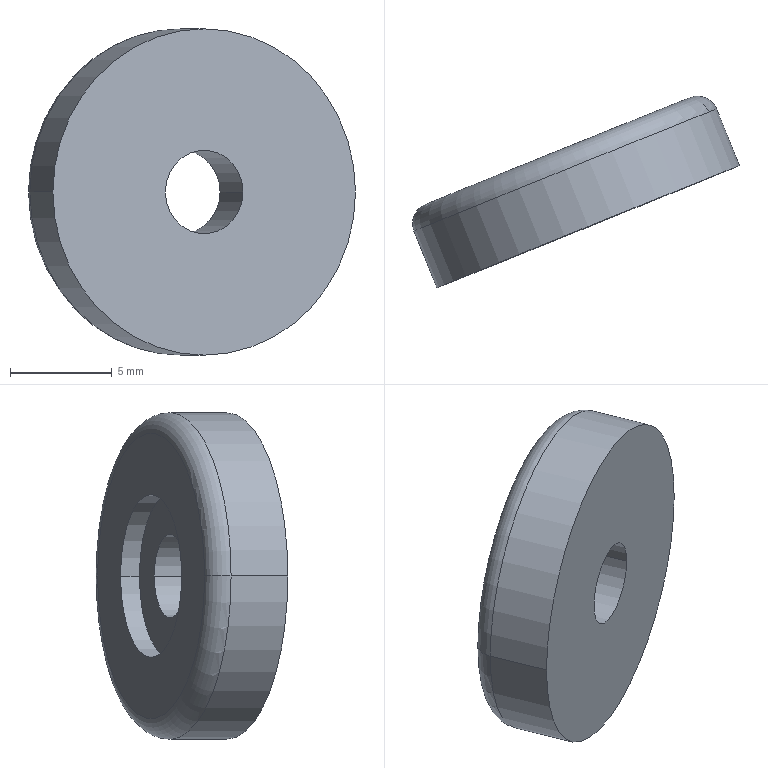Component | SolidWorks | RightDoorAssembly-1_LinkRodLock-1_Roller-4 | 1 solid | 11 faces | box 16.03 x 9.4 x 16 mm | volume 704 mm3 | cylinder 6 | plane 3 | torus 2 | commonest cylinder face diameters 8 x2 16 x2 4.1 x2
build123d program:
from build123d import *

# Parameters (mm, degrees)
SKETCH1_R           = 8
SKETCH1_R_2         = 2.05
BOSS_EXTRUDE1_DEPTH = 4
SKETCH2_R           = 4
CUT_EXTRUDE1_DEPTH  = 1
FILLET1_R           = 1


with BuildPart() as part:
    # Sketch1 → Boss-Extrude1 (new body)
    with BuildSketch(Plane.XY):
        Circle(SKETCH1_R)
        Circle(SKETCH1_R_2, mode=Mode.SUBTRACT)
    extrude(amount=BOSS_EXTRUDE1_DEPTH)

    # Sketch2 → Cut-Extrude1 (cut)
    with BuildSketch(Plane.XY.offset(4)):
        Circle(SKETCH2_R)
    extrude(amount=-CUT_EXTRUDE1_DEPTH, mode=Mode.SUBTRACT)

    # Fillet1
    fillet1_edges = [part.edges().sort_by_distance(p)[0] for p in [
        (-8, 0, 4),
    ]]
    fillet(fillet1_edges, radius=FILLET1_R)


solid = part.part

# Placed as in the assembly
solid = solid.moved(Location((-316.148, 410.532, 94.7), (-90, -21.985, 6.077)))
STEP:
#1=COLOUR_RGB('',0.7922,0.8196,0.9333);
#2=FILL_AREA_STYLE_COLOUR('',#1);
#3=FILL_AREA_STYLE('',(#2));
#4=SURFACE_STYLE_FILL_AREA(#3);
#5=SURFACE_SIDE_STYLE('',(#4));
#6=SURFACE_STYLE_USAGE(.BOTH.,#5);
#7=PRESENTATION_STYLE_ASSIGNMENT((#6));
#8=CARTESIAN_POINT('',(-12.199,16.39,3.728));
#9=VERTEX_POINT('',#8);
#10=CARTESIAN_POINT('',(-12.783,16.154,3.728));
#11=VERTEX_POINT('',#10);
#12=CARTESIAN_POINT('',(-12.491,16.272,3.728));
#13=DIRECTION('',(0.3744,-0.9273,0.));
#14=DIRECTION('',(-0.9273,-0.3744,0.));
#15=AXIS2_PLACEMENT_3D('',#12,#13,#14);
#16=CIRCLE('',#15,0.315);
#17=EDGE_CURVE('',#9,#11,#16,.T.);
#18=ORIENTED_EDGE('',*,*,#17,.F.);
#19=CARTESIAN_POINT('',(-12.25,16.412,3.728));
#20=VERTEX_POINT('',#19);
#21=CARTESIAN_POINT('',(-12.235,16.375,3.728));
#22=DIRECTION('',(0.,0.,1.));
#23=DIRECTION('',(0.,-1.,0.));
#24=AXIS2_PLACEMENT_3D('',#21,#22,#23);
#25=CIRCLE('',#24,0.03937);
#26=EDGE_CURVE('',#9,#20,#25,.T.);
#27=ORIENTED_EDGE('',*,*,#26,.T.);
#28=CARTESIAN_POINT('',(-12.761,16.206,3.728));
#29=VERTEX_POINT('',#28);
#30=CARTESIAN_POINT('',(-12.506,16.309,3.728));
#31=DIRECTION('',(-0.3744,0.9273,-0.));
#32=DIRECTION('',(-0.9273,-0.3744,0.));
#33=AXIS2_PLACEMENT_3D('',#30,#31,#32);
#34=CIRCLE('',#33,0.2756);
#35=EDGE_CURVE('',#29,#20,#34,.T.);
#36=ORIENTED_EDGE('',*,*,#35,.F.);
#37=CARTESIAN_POINT('',(-12.747,16.169,3.728));
#38=DIRECTION('',(-0.,-0.,-1.));
#39=DIRECTION('',(0.,1.,-0.));
#40=AXIS2_PLACEMENT_3D('',#37,#38,#39);
#41=CIRCLE('',#40,0.03937);
#42=EDGE_CURVE('',#11,#29,#41,.T.);
#43=ORIENTED_EDGE('',*,*,#42,.F.);
#44=EDGE_LOOP('',(#18,#27,#36,#43));
#45=FACE_OUTER_BOUND('',#44,.T.);
#46=CARTESIAN_POINT('',(-12.491,16.272,3.728));
#47=DIRECTION('',(-0.3744,0.9273,-0.));
#48=DIRECTION('',(-0.9273,-0.3744,0.));
#49=AXIS2_PLACEMENT_3D('',#46,#47,#48);
#50=TOROIDAL_SURFACE('',#49,0.2756,0.03937);
#51=ADVANCED_FACE('',(#45),#50,.T.);
#52=CARTESIAN_POINT('',(-12.345,16.331,3.728));
#53=VERTEX_POINT('',#52);
#54=CARTESIAN_POINT('',(-12.637,16.213,3.728));
#55=VERTEX_POINT('',#54);
#56=CARTESIAN_POINT('',(-12.491,16.272,3.728));
#57=DIRECTION('',(-0.3744,0.9273,-0.));
#58=DIRECTION('',(-0.9273,-0.3744,0.));
#59=AXIS2_PLACEMENT_3D('',#56,#57,#58);
#60=CIRCLE('',#59,0.1575);
#61=EDGE_CURVE('',#53,#55,#60,.T.);
#62=ORIENTED_EDGE('',*,*,#61,.F.);
#63=CARTESIAN_POINT('',(-12.36,16.368,3.728));
#64=VERTEX_POINT('',#63);
#65=CARTESIAN_POINT('',(-12.345,16.331,3.728));
#66=DIRECTION('',(-0.3744,0.9273,-0.));
#67=VECTOR('',#66,39.37);
#68=LINE('',#65,#67);
#69=EDGE_CURVE('',#53,#64,#68,.T.);
#70=ORIENTED_EDGE('',*,*,#69,.T.);
#71=CARTESIAN_POINT('',(-12.652,16.25,3.728));
#72=VERTEX_POINT('',#71);
#73=CARTESIAN_POINT('',(-12.506,16.309,3.728));
#74=DIRECTION('',(-0.3744,0.9273,-0.));
#75=DIRECTION('',(-0.9273,-0.3744,0.));
#76=AXIS2_PLACEMENT_3D('',#73,#74,#75);
#77=CIRCLE('',#76,0.1575);
#78=EDGE_CURVE('',#64,#72,#77,.T.);
#79=ORIENTED_EDGE('',*,*,#78,.T.);
#80=CARTESIAN_POINT('',(-12.637,16.213,3.728));
#81=DIRECTION('',(-0.3744,0.9273,-0.));
#82=VECTOR('',#81,39.37);
#83=LINE('',#80,#82);
#84=EDGE_CURVE('',#55,#72,#83,.T.);
#85=ORIENTED_EDGE('',*,*,#84,.F.);
#86=EDGE_LOOP('',(#62,#70,#79,#85));
#87=FACE_OUTER_BOUND('',#86,.T.);
#88=CARTESIAN_POINT('',(-12.491,16.272,3.728));
#89=DIRECTION('',(-0.3744,0.9273,-0.));
#90=DIRECTION('',(-0.9273,-0.3744,0.));
#91=AXIS2_PLACEMENT_3D('',#88,#89,#90);
#92=CYLINDRICAL_SURFACE('',#91,0.1575);
#93=ADVANCED_FACE('',(#87),#92,.F.);
#94=ORIENTED_EDGE('',*,*,#17,.T.);
#95=CARTESIAN_POINT('',(-12.739,16.045,3.728));
#96=VERTEX_POINT('',#95);
#97=CARTESIAN_POINT('',(-12.798,16.191,3.728));
#98=DIRECTION('',(0.3744,-0.9273,0.));
#99=VECTOR('',#98,39.37);
#100=LINE('',#97,#99);
#101=EDGE_CURVE('',#11,#96,#100,.T.);
#102=ORIENTED_EDGE('',*,*,#101,.T.);
#103=CARTESIAN_POINT('',(-12.155,16.281,3.728));
#104=VERTEX_POINT('',#103);
#105=CARTESIAN_POINT('',(-12.447,16.163,3.728));
#106=DIRECTION('',(-0.3744,0.9273,-0.));
#107=DIRECTION('',(-0.9273,-0.3744,0.));
#108=AXIS2_PLACEMENT_3D('',#105,#106,#107);
#109=CIRCLE('',#108,0.315);
#110=EDGE_CURVE('',#96,#104,#109,.T.);
#111=ORIENTED_EDGE('',*,*,#110,.T.);
#112=CARTESIAN_POINT('',(-12.214,16.427,3.728));
#113=DIRECTION('',(0.3744,-0.9273,0.));
#114=VECTOR('',#113,39.37);
#115=LINE('',#112,#114);
#116=EDGE_CURVE('',#9,#104,#115,.T.);
#117=ORIENTED_EDGE('',*,*,#116,.F.);
#118=EDGE_LOOP('',(#94,#102,#111,#117));
#119=FACE_OUTER_BOUND('',#118,.T.);
#120=CARTESIAN_POINT('',(-12.506,16.309,3.728));
#121=DIRECTION('',(0.3744,-0.9273,0.));
#122=DIRECTION('',(0.9273,0.3744,-0.));
#123=AXIS2_PLACEMENT_3D('',#120,#121,#122);
#124=CYLINDRICAL_SURFACE('',#123,0.315);
#125=ADVANCED_FACE('',(#119),#124,.T.);
#126=CARTESIAN_POINT('',(-12.416,16.302,3.728));
#127=VERTEX_POINT('',#126);
#128=CARTESIAN_POINT('',(-12.566,16.242,3.728));
#129=VERTEX_POINT('',#128);
#130=CARTESIAN_POINT('',(-12.491,16.272,3.728));
#131=DIRECTION('',(-0.3744,0.9273,-0.));
#132=DIRECTION('',(-0.9273,-0.3744,0.));
#133=AXIS2_PLACEMENT_3D('',#130,#131,#132);
#134=CIRCLE('',#133,0.08071);
#135=EDGE_CURVE('',#127,#129,#134,.T.);
#136=ORIENTED_EDGE('',*,*,#135,.T.);
#137=CARTESIAN_POINT('',(-12.522,16.132,3.728));
#138=VERTEX_POINT('',#137);
#139=CARTESIAN_POINT('',(-12.581,16.278,3.728));
#140=DIRECTION('',(0.3744,-0.9273,0.));
#141=VECTOR('',#140,39.37);
#142=LINE('',#139,#141);
#143=EDGE_CURVE('',#129,#138,#142,.T.);
#144=ORIENTED_EDGE('',*,*,#143,.T.);
#145=CARTESIAN_POINT('',(-12.372,16.193,3.728));
#146=VERTEX_POINT('',#145);
#147=CARTESIAN_POINT('',(-12.447,16.163,3.728));
#148=DIRECTION('',(-0.3744,0.9273,-0.));
#149=DIRECTION('',(-0.9273,-0.3744,0.));
#150=AXIS2_PLACEMENT_3D('',#147,#148,#149);
#151=CIRCLE('',#150,0.08071);
#152=EDGE_CURVE('',#146,#138,#151,.T.);
#153=ORIENTED_EDGE('',*,*,#152,.F.);
#154=CARTESIAN_POINT('',(-12.431,16.339,3.728));
#155=DIRECTION('',(0.3744,-0.9273,0.));
#156=VECTOR('',#155,39.37);
#157=LINE('',#154,#156);
#158=EDGE_CURVE('',#127,#146,#157,.T.);
#159=ORIENTED_EDGE('',*,*,#158,.F.);
#160=EDGE_LOOP('',(#136,#144,#153,#159));
#161=FACE_OUTER_BOUND('',#160,.T.);
#162=CARTESIAN_POINT('',(-12.506,16.309,3.728));
#163=DIRECTION('',(0.3744,-0.9273,0.));
#164=DIRECTION('',(0.9273,0.3744,-0.));
#165=AXIS2_PLACEMENT_3D('',#162,#163,#164);
#166=CYLINDRICAL_SURFACE('',#165,0.08071);
#167=ADVANCED_FACE('',(#161),#166,.F.);
#168=ORIENTED_EDGE('',*,*,#143,.F.);
#169=CARTESIAN_POINT('',(-12.491,16.272,3.728));
#170=DIRECTION('',(-0.3744,0.9273,-0.));
#171=DIRECTION('',(-0.9273,-0.3744,0.));
#172=AXIS2_PLACEMENT_3D('',#169,#170,#171);
#173=CIRCLE('',#172,0.08071);
#174=EDGE_CURVE('',#129,#127,#173,.T.);
#175=ORIENTED_EDGE('',*,*,#174,.T.);
#176=ORIENTED_EDGE('',*,*,#158,.T.);
#177=CARTESIAN_POINT('',(-12.447,16.163,3.728));
#178=DIRECTION('',(-0.3744,0.9273,-0.));
#179=DIRECTION('',(-0.9273,-0.3744,0.));
#180=AXIS2_PLACEMENT_3D('',#177,#178,#179);
#181=CIRCLE('',#180,0.08071);
#182=EDGE_CURVE('',#138,#146,#181,.T.);
#183=ORIENTED_EDGE('',*,*,#182,.F.);
#184=EDGE_LOOP('',(#168,#175,#176,#183));
#185=FACE_OUTER_BOUND('',#184,.T.);
#186=CARTESIAN_POINT('',(-12.506,16.309,3.728));
#187=DIRECTION('',(0.3744,-0.9273,0.));
#188=DIRECTION('',(0.9273,0.3744,-0.));
#189=AXIS2_PLACEMENT_3D('',#186,#187,#188);
#190=CYLINDRICAL_SURFACE('',#189,0.08071);
#191=ADVANCED_FACE('',(#185),#190,.F.);
#192=ORIENTED_EDGE('',*,*,#35,.T.);
#193=CARTESIAN_POINT('',(-12.506,16.309,3.728));
#194=DIRECTION('',(-0.3744,0.9273,-0.));
#195=DIRECTION('',(-0.9273,-0.3744,0.));
#196=AXIS2_PLACEMENT_3D('',#193,#194,#195);
#197=CIRCLE('',#196,0.2756);
#198=EDGE_CURVE('',#20,#29,#197,.T.);
#199=ORIENTED_EDGE('',*,*,#198,.T.);
#200=EDGE_LOOP('',(#192,#199));
#201=FACE_OUTER_BOUND('',#200,.T.);
#202=CARTESIAN_POINT('',(-12.506,16.309,3.728));
#203=DIRECTION('',(-0.3744,0.9273,-0.));
#204=DIRECTION('',(-0.9273,-0.3744,0.));
#205=AXIS2_PLACEMENT_3D('',#202,#203,#204);
#206=CIRCLE('',#205,0.1575);
#207=EDGE_CURVE('',#72,#64,#206,.T.);
#208=ORIENTED_EDGE('',*,*,#207,.F.);
#209=ORIENTED_EDGE('',*,*,#78,.F.);
#210=EDGE_LOOP('',(#208,#209));
#211=FACE_BOUND('',#210,.T.);
#212=CARTESIAN_POINT('',(-12.506,16.309,3.728));
#213=DIRECTION('',(-0.3744,0.9273,-0.));
#214=DIRECTION('',(-0.9273,-0.3744,0.));
#215=AXIS2_PLACEMENT_3D('',#212,#213,#214);
#216=PLANE('',#215);
#217=ADVANCED_FACE('',(#201,#211),#216,.T.);
#218=CARTESIAN_POINT('',(-12.447,16.163,3.728));
#219=DIRECTION('',(-0.3744,0.9273,-0.));
#220=DIRECTION('',(-0.9273,-0.3744,0.));
#221=AXIS2_PLACEMENT_3D('',#218,#219,#220);
#222=CIRCLE('',#221,0.315);
#223=EDGE_CURVE('',#104,#96,#222,.T.);
#224=ORIENTED_EDGE('',*,*,#223,.F.);
#225=ORIENTED_EDGE('',*,*,#110,.F.);
#226=EDGE_LOOP('',(#224,#225));
#227=FACE_OUTER_BOUND('',#226,.T.);
#228=ORIENTED_EDGE('',*,*,#152,.T.);
#229=ORIENTED_EDGE('',*,*,#182,.T.);
#230=EDGE_LOOP('',(#228,#229));
#231=FACE_BOUND('',#230,.T.);
#232=CARTESIAN_POINT('',(-12.447,16.163,3.728));
#233=DIRECTION('',(-0.3744,0.9273,-0.));
#234=DIRECTION('',(-0.9273,-0.3744,0.));
#235=AXIS2_PLACEMENT_3D('',#232,#233,#234);
#236=PLANE('',#235);
#237=ADVANCED_FACE('',(#227,#231),#236,.F.);
#238=ORIENTED_EDGE('',*,*,#101,.F.);
#239=CARTESIAN_POINT('',(-12.491,16.272,3.728));
#240=DIRECTION('',(0.3744,-0.9273,0.));
#241=DIRECTION('',(-0.9273,-0.3744,0.));
#242=AXIS2_PLACEMENT_3D('',#239,#240,#241);
#243=CIRCLE('',#242,0.315);
#244=EDGE_CURVE('',#11,#9,#243,.T.);
#245=ORIENTED_EDGE('',*,*,#244,.T.);
#246=ORIENTED_EDGE('',*,*,#116,.T.);
#247=ORIENTED_EDGE('',*,*,#223,.T.);
#248=EDGE_LOOP('',(#238,#245,#246,#247));
#249=FACE_OUTER_BOUND('',#248,.T.);
#250=CARTESIAN_POINT('',(-12.506,16.309,3.728));
#251=DIRECTION('',(0.3744,-0.9273,0.));
#252=DIRECTION('',(0.9273,0.3744,-0.));
#253=AXIS2_PLACEMENT_3D('',#250,#251,#252);
#254=CYLINDRICAL_SURFACE('',#253,0.315);
#255=ADVANCED_FACE('',(#249),#254,.T.);
#256=ORIENTED_EDGE('',*,*,#69,.F.);
#257=CARTESIAN_POINT('',(-12.491,16.272,3.728));
#258=DIRECTION('',(-0.3744,0.9273,-0.));
#259=DIRECTION('',(-0.9273,-0.3744,0.));
#260=AXIS2_PLACEMENT_3D('',#257,#258,#259);
#261=CIRCLE('',#260,0.1575);
#262=EDGE_CURVE('',#55,#53,#261,.T.);
#263=ORIENTED_EDGE('',*,*,#262,.F.);
#264=ORIENTED_EDGE('',*,*,#84,.T.);
#265=ORIENTED_EDGE('',*,*,#207,.T.);
#266=EDGE_LOOP('',(#256,#263,#264,#265));
#267=FACE_OUTER_BOUND('',#266,.T.);
#268=CARTESIAN_POINT('',(-12.491,16.272,3.728));
#269=DIRECTION('',(-0.3744,0.9273,-0.));
#270=DIRECTION('',(-0.9273,-0.3744,0.));
#271=AXIS2_PLACEMENT_3D('',#268,#269,#270);
#272=CYLINDRICAL_SURFACE('',#271,0.1575);
#273=ADVANCED_FACE('',(#267),#272,.F.);
#274=ORIENTED_EDGE('',*,*,#135,.F.);
#275=ORIENTED_EDGE('',*,*,#174,.F.);
#276=EDGE_LOOP('',(#274,#275));
#277=FACE_BOUND('',#276,.T.);
#278=ORIENTED_EDGE('',*,*,#262,.T.);
#279=ORIENTED_EDGE('',*,*,#61,.T.);
#280=EDGE_LOOP('',(#278,#279));
#281=FACE_OUTER_BOUND('',#280,.T.);
#282=CARTESIAN_POINT('',(-12.491,16.272,3.728));
#283=DIRECTION('',(-0.3744,0.9273,-0.));
#284=DIRECTION('',(-0.9273,-0.3744,0.));
#285=AXIS2_PLACEMENT_3D('',#282,#283,#284);
#286=PLANE('',#285);
#287=ADVANCED_FACE('',(#277,#281),#286,.T.);
#288=ORIENTED_EDGE('',*,*,#26,.F.);
#289=ORIENTED_EDGE('',*,*,#244,.F.);
#290=ORIENTED_EDGE('',*,*,#42,.T.);
#291=ORIENTED_EDGE('',*,*,#198,.F.);
#292=EDGE_LOOP('',(#288,#289,#290,#291));
#293=FACE_OUTER_BOUND('',#292,.T.);
#294=CARTESIAN_POINT('',(-12.491,16.272,3.728));
#295=DIRECTION('',(-0.3744,0.9273,-0.));
#296=DIRECTION('',(-0.9273,-0.3744,0.));
#297=AXIS2_PLACEMENT_3D('',#294,#295,#296);
#298=TOROIDAL_SURFACE('',#297,0.2756,0.03937);
#299=ADVANCED_FACE('',(#293),#298,.T.);
#300=CLOSED_SHELL('',(#51,#93,#125,#167,#191,#217,#237,#255,#273,#287,#299));
#301=MANIFOLD_SOLID_BREP('',#300);
#302=STYLED_ITEM('',(#7),#301);
#303=(LENGTH_UNIT()NAMED_UNIT(*)SI_UNIT($,.METRE.));
#304=LENGTH_MEASURE_WITH_UNIT(LENGTH_MEASURE(0.0254),#303);
#305=DIMENSIONAL_EXPONENTS(1.,0.,0.,0.,0.,0.,0.);
#306=(CONVERSION_BASED_UNIT('',#304)LENGTH_UNIT()NAMED_UNIT(#305));
#307=UNCERTAINTY_MEASURE_WITH_UNIT(LENGTH_MEASURE(0.00001),#306,'','');
#308=(NAMED_UNIT(*)PLANE_ANGLE_UNIT()SI_UNIT($,.RADIAN.));
#309=(NAMED_UNIT(*)SI_UNIT($,.STERADIAN.)SOLID_ANGLE_UNIT());
#310=(GEOMETRIC_REPRESENTATION_CONTEXT(3)GLOBAL_UNCERTAINTY_ASSIGNED_CONTEXT((#307))GLOBAL_UNIT_ASSIGNED_CONTEXT((#306,#308,#309))REPRESENTATION_CONTEXT('',''));
#311=MECHANICAL_DESIGN_GEOMETRIC_PRESENTATION_REPRESENTATION('',(#302),#310);
#312=CARTESIAN_POINT('',(0.,0.,0.));
#313=DIRECTION('',(0.,0.,1.));
#314=DIRECTION('',(1.,0.,0.));
#315=AXIS2_PLACEMENT_3D('',#312,#313,#314);
#316=(LENGTH_UNIT()NAMED_UNIT(*)SI_UNIT($,.METRE.));
#317=LENGTH_MEASURE_WITH_UNIT(LENGTH_MEASURE(0.0254),#316);
#318=DIMENSIONAL_EXPONENTS(1.,0.,0.,0.,0.,0.,0.);
#319=(CONVERSION_BASED_UNIT('',#317)LENGTH_UNIT()NAMED_UNIT(#318));
#320=UNCERTAINTY_MEASURE_WITH_UNIT(LENGTH_MEASURE(0.00001),#319,'','');
#321=(NAMED_UNIT(*)PLANE_ANGLE_UNIT()SI_UNIT($,.RADIAN.));
#322=(NAMED_UNIT(*)SI_UNIT($,.STERADIAN.)SOLID_ANGLE_UNIT());
#323=(GEOMETRIC_REPRESENTATION_CONTEXT(3)GLOBAL_UNCERTAINTY_ASSIGNED_CONTEXT((#320))GLOBAL_UNIT_ASSIGNED_CONTEXT((#319,#321,#322))REPRESENTATION_CONTEXT('',''));
#324=ADVANCED_BREP_SHAPE_REPRESENTATION('',(#301,#315),#323);
#325=PRESENTATION_LAYER_ASSIGNMENT('','',(#302));